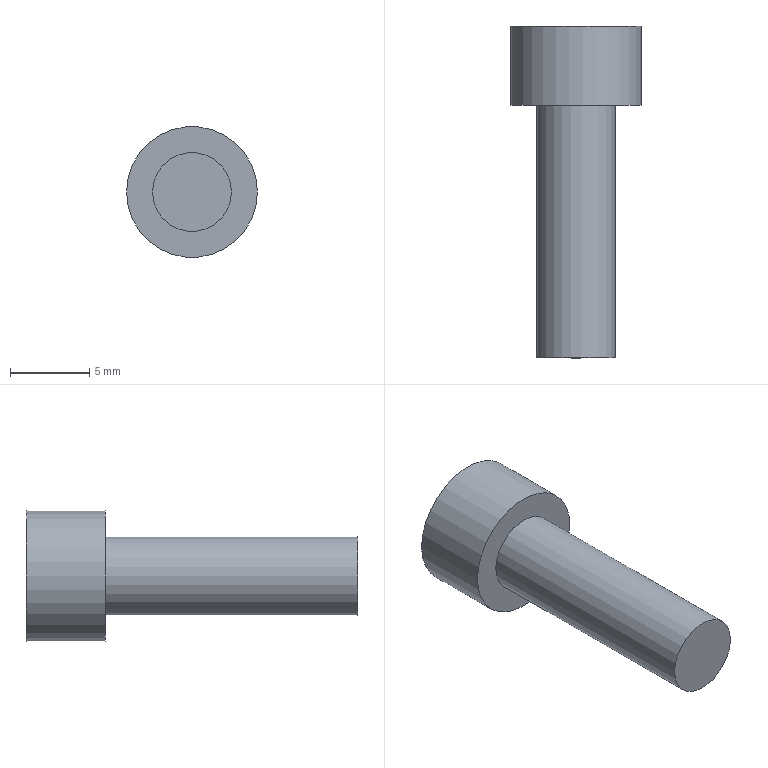Component | NX | HEX_SCREW_M5_16 | 1 solid | 12 faces | box 8.28 x 21 x 8.28 mm | volume 549 mm3 | plane 10 | cylinder 2 | commonest cylinder face diameters 8.28 x1 5 x1
STEP:
#1=CARTESIAN_POINT('',(0.,0.,0.));
#2=DIRECTION('',(0.,0.,1.));
#3=DIRECTION('',(1.,0.,0.));
#4=AXIS2_PLACEMENT_3D('',#1,#2,#3);
#5=CARTESIAN_POINT('',(26.14,-6.7,44.));
#6=VERTEX_POINT('',#5);
#7=CARTESIAN_POINT('',(22.,-6.7,44.));
#8=DIRECTION('',(0.,1.,0.));
#9=DIRECTION('',(1.,0.,0.));
#10=AXIS2_PLACEMENT_3D('',#7,#8,#9);
#11=CIRCLE('',#10,4.14);
#12=CARTESIAN_POINT('',(22.,-6.7,44.));
#13=DIRECTION('',(0.,1.,0.));
#14=DIRECTION('',(-1.,0.,0.));
#15=AXIS2_PLACEMENT_3D('',#12,#13,#14);
#16=PLANE('',#15);
#17=CARTESIAN_POINT('',(0.,0.));
#18=DIRECTION('',(-1.,0.));
#19=AXIS2_PLACEMENT_2D('',#17,#18);
#20=CIRCLE('',#19,4.14);
#21=(GEOMETRIC_REPRESENTATION_CONTEXT(2)PARAMETRIC_REPRESENTATION_CONTEXT()REPRESENTATION_CONTEXT('',''));
#22=DEFINITIONAL_REPRESENTATION('',(#20),#21);
#23=PCURVE('',#16,#22);
#24=CARTESIAN_POINT('',(22.,-11.7,44.));
#25=DIRECTION('',(0.,1.,0.));
#26=DIRECTION('',(-1.,0.,0.));
#27=AXIS2_PLACEMENT_3D('',#24,#25,#26);
#28=CYLINDRICAL_SURFACE('',#27,4.14);
#29=CARTESIAN_POINT('',(3.142,5.));
#30=DIRECTION('',(1.,0.));
#31=VECTOR('',#30,1.);
#32=LINE('',#29,#31);
#33=(GEOMETRIC_REPRESENTATION_CONTEXT(2)PARAMETRIC_REPRESENTATION_CONTEXT()REPRESENTATION_CONTEXT('',''));
#34=DEFINITIONAL_REPRESENTATION('',(#32),#33);
#35=PCURVE('',#28,#34);
#36=SURFACE_CURVE('',#11,(#23,#35),.PCURVE_S1.);
#37=EDGE_CURVE('',#6,#6,#36,.T.);
#38=ORIENTED_EDGE('',*,*,#37,.T.);
#39=EDGE_LOOP('',(#38));
#40=FACE_BOUND('',#39,.T.);
#41=CARTESIAN_POINT('',(22.,-6.7,41.691));
#42=VERTEX_POINT('',#41);
#43=CARTESIAN_POINT('',(24.,-6.7,42.845));
#44=VERTEX_POINT('',#43);
#45=CARTESIAN_POINT('',(22.,-6.7,41.691));
#46=DIRECTION('',(0.866,0.,0.5));
#47=VECTOR('',#46,1.);
#48=LINE('',#45,#47);
#49=CARTESIAN_POINT('',(0.,-2.309));
#50=DIRECTION('',(-0.866,0.5));
#51=VECTOR('',#50,1.);
#52=LINE('',#49,#51);
#53=(GEOMETRIC_REPRESENTATION_CONTEXT(2)PARAMETRIC_REPRESENTATION_CONTEXT()REPRESENTATION_CONTEXT('',''));
#54=DEFINITIONAL_REPRESENTATION('',(#52),#53);
#55=PCURVE('',#16,#54);
#56=CARTESIAN_POINT('',(22.,-9.2,41.691));
#57=DIRECTION('',(-0.5,0.,0.866));
#58=DIRECTION('',(-0.866,0.,-0.5));
#59=AXIS2_PLACEMENT_3D('',#56,#57,#58);
#60=PLANE('',#59);
#61=CARTESIAN_POINT('',(0.,-2.5));
#62=DIRECTION('',(-1.,0.));
#63=VECTOR('',#62,1.);
#64=LINE('',#61,#63);
#65=(GEOMETRIC_REPRESENTATION_CONTEXT(2)PARAMETRIC_REPRESENTATION_CONTEXT()REPRESENTATION_CONTEXT('',''));
#66=DEFINITIONAL_REPRESENTATION('',(#64),#65);
#67=PCURVE('',#60,#66);
#68=SURFACE_CURVE('',#48,(#55,#67),.PCURVE_S1.);
#69=EDGE_CURVE('',#42,#44,#68,.T.);
#70=ORIENTED_EDGE('',*,*,#69,.T.);
#71=CARTESIAN_POINT('',(24.,-6.7,45.155));
#72=VERTEX_POINT('',#71);
#73=CARTESIAN_POINT('',(24.,-6.7,42.845));
#74=DIRECTION('',(0.,0.,1.));
#75=VECTOR('',#74,1.);
#76=LINE('',#73,#75);
#77=CARTESIAN_POINT('',(-2.,-1.155));
#78=DIRECTION('',(0.,1.));
#79=VECTOR('',#78,1.);
#80=LINE('',#77,#79);
#81=(GEOMETRIC_REPRESENTATION_CONTEXT(2)PARAMETRIC_REPRESENTATION_CONTEXT()REPRESENTATION_CONTEXT('',''));
#82=DEFINITIONAL_REPRESENTATION('',(#80),#81);
#83=PCURVE('',#16,#82);
#84=CARTESIAN_POINT('',(24.,-9.2,42.845));
#85=DIRECTION('',(-1.,0.,0.));
#86=DIRECTION('',(0.,-1.,0.));
#87=AXIS2_PLACEMENT_3D('',#84,#85,#86);
#88=PLANE('',#87);
#89=CARTESIAN_POINT('',(-2.5,0.));
#90=DIRECTION('',(0.,1.));
#91=VECTOR('',#90,1.);
#92=LINE('',#89,#91);
#93=(GEOMETRIC_REPRESENTATION_CONTEXT(2)PARAMETRIC_REPRESENTATION_CONTEXT()REPRESENTATION_CONTEXT('',''));
#94=DEFINITIONAL_REPRESENTATION('',(#92),#93);
#95=PCURVE('',#88,#94);
#96=SURFACE_CURVE('',#76,(#83,#95),.PCURVE_S1.);
#97=EDGE_CURVE('',#44,#72,#96,.T.);
#98=ORIENTED_EDGE('',*,*,#97,.T.);
#99=CARTESIAN_POINT('',(22.,-6.7,46.309));
#100=VERTEX_POINT('',#99);
#101=CARTESIAN_POINT('',(24.,-6.7,45.155));
#102=DIRECTION('',(-0.866,0.,0.5));
#103=VECTOR('',#102,1.);
#104=LINE('',#101,#103);
#105=CARTESIAN_POINT('',(-2.,1.155));
#106=DIRECTION('',(0.866,0.5));
#107=VECTOR('',#106,1.);
#108=LINE('',#105,#107);
#109=(GEOMETRIC_REPRESENTATION_CONTEXT(2)PARAMETRIC_REPRESENTATION_CONTEXT()REPRESENTATION_CONTEXT('',''));
#110=DEFINITIONAL_REPRESENTATION('',(#108),#109);
#111=PCURVE('',#16,#110);
#112=CARTESIAN_POINT('',(24.,-9.2,45.155));
#113=DIRECTION('',(-0.5,0.,-0.866));
#114=DIRECTION('',(0.866,0.,-0.5));
#115=AXIS2_PLACEMENT_3D('',#112,#113,#114);
#116=PLANE('',#115);
#117=CARTESIAN_POINT('',(0.,-2.5));
#118=DIRECTION('',(-1.,0.));
#119=VECTOR('',#118,1.);
#120=LINE('',#117,#119);
#121=(GEOMETRIC_REPRESENTATION_CONTEXT(2)PARAMETRIC_REPRESENTATION_CONTEXT()REPRESENTATION_CONTEXT('',''));
#122=DEFINITIONAL_REPRESENTATION('',(#120),#121);
#123=PCURVE('',#116,#122);
#124=SURFACE_CURVE('',#104,(#111,#123),.PCURVE_S1.);
#125=EDGE_CURVE('',#72,#100,#124,.T.);
#126=ORIENTED_EDGE('',*,*,#125,.T.);
#127=CARTESIAN_POINT('',(20.,-6.7,45.155));
#128=VERTEX_POINT('',#127);
#129=CARTESIAN_POINT('',(22.,-6.7,46.309));
#130=DIRECTION('',(-0.866,0.,-0.5));
#131=VECTOR('',#130,1.);
#132=LINE('',#129,#131);
#133=CARTESIAN_POINT('',(0.,2.309));
#134=DIRECTION('',(0.866,-0.5));
#135=VECTOR('',#134,1.);
#136=LINE('',#133,#135);
#137=(GEOMETRIC_REPRESENTATION_CONTEXT(2)PARAMETRIC_REPRESENTATION_CONTEXT()REPRESENTATION_CONTEXT('',''));
#138=DEFINITIONAL_REPRESENTATION('',(#136),#137);
#139=PCURVE('',#16,#138);
#140=CARTESIAN_POINT('',(22.,-9.2,46.309));
#141=DIRECTION('',(0.5,0.,-0.866));
#142=DIRECTION('',(0.866,0.,0.5));
#143=AXIS2_PLACEMENT_3D('',#140,#141,#142);
#144=PLANE('',#143);
#145=CARTESIAN_POINT('',(0.,-2.5));
#146=DIRECTION('',(-1.,0.));
#147=VECTOR('',#146,1.);
#148=LINE('',#145,#147);
#149=(GEOMETRIC_REPRESENTATION_CONTEXT(2)PARAMETRIC_REPRESENTATION_CONTEXT()REPRESENTATION_CONTEXT('',''));
#150=DEFINITIONAL_REPRESENTATION('',(#148),#149);
#151=PCURVE('',#144,#150);
#152=SURFACE_CURVE('',#132,(#139,#151),.PCURVE_S1.);
#153=EDGE_CURVE('',#100,#128,#152,.T.);
#154=ORIENTED_EDGE('',*,*,#153,.T.);
#155=CARTESIAN_POINT('',(20.,-6.7,42.845));
#156=VERTEX_POINT('',#155);
#157=CARTESIAN_POINT('',(20.,-6.7,45.155));
#158=DIRECTION('',(0.,0.,-1.));
#159=VECTOR('',#158,1.);
#160=LINE('',#157,#159);
#161=CARTESIAN_POINT('',(2.,1.155));
#162=DIRECTION('',(0.,-1.));
#163=VECTOR('',#162,1.);
#164=LINE('',#161,#163);
#165=(GEOMETRIC_REPRESENTATION_CONTEXT(2)PARAMETRIC_REPRESENTATION_CONTEXT()REPRESENTATION_CONTEXT('',''));
#166=DEFINITIONAL_REPRESENTATION('',(#164),#165);
#167=PCURVE('',#16,#166);
#168=CARTESIAN_POINT('',(20.,-9.2,45.155));
#169=DIRECTION('',(1.,0.,0.));
#170=DIRECTION('',(0.,1.,0.));
#171=AXIS2_PLACEMENT_3D('',#168,#169,#170);
#172=PLANE('',#171);
#173=CARTESIAN_POINT('',(2.5,0.));
#174=DIRECTION('',(0.,-1.));
#175=VECTOR('',#174,1.);
#176=LINE('',#173,#175);
#177=(GEOMETRIC_REPRESENTATION_CONTEXT(2)PARAMETRIC_REPRESENTATION_CONTEXT()REPRESENTATION_CONTEXT('',''));
#178=DEFINITIONAL_REPRESENTATION('',(#176),#177);
#179=PCURVE('',#172,#178);
#180=SURFACE_CURVE('',#160,(#167,#179),.PCURVE_S1.);
#181=EDGE_CURVE('',#128,#156,#180,.T.);
#182=ORIENTED_EDGE('',*,*,#181,.T.);
#183=CARTESIAN_POINT('',(20.,-6.7,42.845));
#184=DIRECTION('',(0.866,0.,-0.5));
#185=VECTOR('',#184,1.);
#186=LINE('',#183,#185);
#187=CARTESIAN_POINT('',(2.,-1.155));
#188=DIRECTION('',(-0.866,-0.5));
#189=VECTOR('',#188,1.);
#190=LINE('',#187,#189);
#191=(GEOMETRIC_REPRESENTATION_CONTEXT(2)PARAMETRIC_REPRESENTATION_CONTEXT()REPRESENTATION_CONTEXT('',''));
#192=DEFINITIONAL_REPRESENTATION('',(#190),#191);
#193=PCURVE('',#16,#192);
#194=CARTESIAN_POINT('',(20.,-9.2,42.845));
#195=DIRECTION('',(0.5,0.,0.866));
#196=DIRECTION('',(-0.866,0.,0.5));
#197=AXIS2_PLACEMENT_3D('',#194,#195,#196);
#198=PLANE('',#197);
#199=CARTESIAN_POINT('',(0.,-2.5));
#200=DIRECTION('',(-1.,0.));
#201=VECTOR('',#200,1.);
#202=LINE('',#199,#201);
#203=(GEOMETRIC_REPRESENTATION_CONTEXT(2)PARAMETRIC_REPRESENTATION_CONTEXT()REPRESENTATION_CONTEXT('',''));
#204=DEFINITIONAL_REPRESENTATION('',(#202),#203);
#205=PCURVE('',#198,#204);
#206=SURFACE_CURVE('',#186,(#193,#205),.PCURVE_S1.);
#207=EDGE_CURVE('',#156,#42,#206,.T.);
#208=ORIENTED_EDGE('',*,*,#207,.T.);
#209=EDGE_LOOP('',(#70,#98,#126,#154,#182,#208));
#210=FACE_BOUND('',#209,.T.);
#211=ADVANCED_FACE('',(#40,#210),#16,.T.);
#212=CARTESIAN_POINT('',(26.14,-11.7,44.));
#213=VERTEX_POINT('',#212);
#214=CARTESIAN_POINT('',(22.,-11.7,44.));
#215=DIRECTION('',(0.,1.,0.));
#216=DIRECTION('',(1.,0.,0.));
#217=AXIS2_PLACEMENT_3D('',#214,#215,#216);
#218=CIRCLE('',#217,4.14);
#219=CARTESIAN_POINT('',(3.142,0.));
#220=DIRECTION('',(1.,0.));
#221=VECTOR('',#220,1.);
#222=LINE('',#219,#221);
#223=(GEOMETRIC_REPRESENTATION_CONTEXT(2)PARAMETRIC_REPRESENTATION_CONTEXT()REPRESENTATION_CONTEXT('',''));
#224=DEFINITIONAL_REPRESENTATION('',(#222),#223);
#225=PCURVE('',#28,#224);
#226=CARTESIAN_POINT('',(22.,-11.7,44.));
#227=DIRECTION('',(0.,1.,0.));
#228=DIRECTION('',(-1.,0.,0.));
#229=AXIS2_PLACEMENT_3D('',#226,#227,#228);
#230=PLANE('',#229);
#231=CARTESIAN_POINT('',(0.,0.));
#232=DIRECTION('',(-1.,0.));
#233=AXIS2_PLACEMENT_2D('',#231,#232);
#234=CIRCLE('',#233,4.14);
#235=(GEOMETRIC_REPRESENTATION_CONTEXT(2)PARAMETRIC_REPRESENTATION_CONTEXT()REPRESENTATION_CONTEXT('',''));
#236=DEFINITIONAL_REPRESENTATION('',(#234),#235);
#237=PCURVE('',#230,#236);
#238=SURFACE_CURVE('',#218,(#225,#237),.PCURVE_S1.);
#239=EDGE_CURVE('',#213,#213,#238,.T.);
#240=ORIENTED_EDGE('',*,*,#239,.T.);
#241=CARTESIAN_POINT('',(26.14,-11.7,44.));
#242=CARTESIAN_POINT('',(26.14,-6.7,44.));
#243=B_SPLINE_CURVE_WITH_KNOTS('',1,(#241,#242),.UNSPECIFIED.,.F.,.F.,(2,2),(0.,5.),.PIECEWISE_BEZIER_KNOTS.);
#244=CARTESIAN_POINT('',(9.425,0.));
#245=DIRECTION('',(0.,1.));
#246=VECTOR('',#245,1.);
#247=LINE('',#244,#246);
#248=(GEOMETRIC_REPRESENTATION_CONTEXT(2)PARAMETRIC_REPRESENTATION_CONTEXT()REPRESENTATION_CONTEXT('',''));
#249=DEFINITIONAL_REPRESENTATION('',(#247),#248);
#250=PCURVE('',#28,#249);
#251=CARTESIAN_POINT('',(3.142,0.));
#252=DIRECTION('',(0.,1.));
#253=VECTOR('',#252,1.);
#254=LINE('',#251,#253);
#255=(GEOMETRIC_REPRESENTATION_CONTEXT(2)PARAMETRIC_REPRESENTATION_CONTEXT()REPRESENTATION_CONTEXT('',''));
#256=DEFINITIONAL_REPRESENTATION('',(#254),#255);
#257=PCURVE('',#28,#256);
#258=SEAM_CURVE('',#243,(#250,#257),.PCURVE_S1.);
#259=EDGE_CURVE('',#213,#6,#258,.T.);
#260=ORIENTED_EDGE('',*,*,#259,.T.);
#261=ORIENTED_EDGE('',*,*,#37,.F.);
#262=ORIENTED_EDGE('',*,*,#259,.F.);
#263=EDGE_LOOP('',(#240,#260,#261,#262));
#264=FACE_BOUND('',#263,.T.);
#265=ADVANCED_FACE('',(#264),#28,.T.);
#266=CARTESIAN_POINT('',(24.5,-11.7,44.));
#267=VERTEX_POINT('',#266);
#268=CARTESIAN_POINT('',(22.,-11.7,44.));
#269=DIRECTION('',(0.,1.,0.));
#270=DIRECTION('',(1.,0.,0.));
#271=AXIS2_PLACEMENT_3D('',#268,#269,#270);
#272=CIRCLE('',#271,2.5);
#273=CARTESIAN_POINT('',(0.,0.));
#274=DIRECTION('',(-1.,0.));
#275=AXIS2_PLACEMENT_2D('',#273,#274);
#276=CIRCLE('',#275,2.5);
#277=(GEOMETRIC_REPRESENTATION_CONTEXT(2)PARAMETRIC_REPRESENTATION_CONTEXT()REPRESENTATION_CONTEXT('',''));
#278=DEFINITIONAL_REPRESENTATION('',(#276),#277);
#279=PCURVE('',#230,#278);
#280=CARTESIAN_POINT('',(22.,-27.7,44.));
#281=DIRECTION('',(0.,1.,0.));
#282=DIRECTION('',(-1.,0.,0.));
#283=AXIS2_PLACEMENT_3D('',#280,#281,#282);
#284=CYLINDRICAL_SURFACE('',#283,2.5);
#285=CARTESIAN_POINT('',(3.142,16.));
#286=DIRECTION('',(1.,0.));
#287=VECTOR('',#286,1.);
#288=LINE('',#285,#287);
#289=(GEOMETRIC_REPRESENTATION_CONTEXT(2)PARAMETRIC_REPRESENTATION_CONTEXT()REPRESENTATION_CONTEXT('',''));
#290=DEFINITIONAL_REPRESENTATION('',(#288),#289);
#291=PCURVE('',#284,#290);
#292=SURFACE_CURVE('',#272,(#279,#291),.PCURVE_S1.);
#293=EDGE_CURVE('',#267,#267,#292,.T.);
#294=ORIENTED_EDGE('',*,*,#293,.T.);
#295=EDGE_LOOP('',(#294));
#296=FACE_BOUND('',#295,.T.);
#297=ORIENTED_EDGE('',*,*,#239,.F.);
#298=EDGE_LOOP('',(#297));
#299=FACE_BOUND('',#298,.T.);
#300=ADVANCED_FACE('',(#296,#299),#230,.F.);
#301=CARTESIAN_POINT('',(24.5,-27.7,44.));
#302=VERTEX_POINT('',#301);
#303=CARTESIAN_POINT('',(22.,-27.7,44.));
#304=DIRECTION('',(0.,1.,0.));
#305=DIRECTION('',(1.,0.,0.));
#306=AXIS2_PLACEMENT_3D('',#303,#304,#305);
#307=CIRCLE('',#306,2.5);
#308=CARTESIAN_POINT('',(3.142,0.));
#309=DIRECTION('',(1.,0.));
#310=VECTOR('',#309,1.);
#311=LINE('',#308,#310);
#312=(GEOMETRIC_REPRESENTATION_CONTEXT(2)PARAMETRIC_REPRESENTATION_CONTEXT()REPRESENTATION_CONTEXT('',''));
#313=DEFINITIONAL_REPRESENTATION('',(#311),#312);
#314=PCURVE('',#284,#313);
#315=CARTESIAN_POINT('',(22.,-27.7,44.));
#316=DIRECTION('',(0.,1.,0.));
#317=DIRECTION('',(-1.,0.,0.));
#318=AXIS2_PLACEMENT_3D('',#315,#316,#317);
#319=PLANE('',#318);
#320=CARTESIAN_POINT('',(0.,0.));
#321=DIRECTION('',(-1.,0.));
#322=AXIS2_PLACEMENT_2D('',#320,#321);
#323=CIRCLE('',#322,2.5);
#324=(GEOMETRIC_REPRESENTATION_CONTEXT(2)PARAMETRIC_REPRESENTATION_CONTEXT()REPRESENTATION_CONTEXT('',''));
#325=DEFINITIONAL_REPRESENTATION('',(#323),#324);
#326=PCURVE('',#319,#325);
#327=SURFACE_CURVE('',#307,(#314,#326),.PCURVE_S1.);
#328=EDGE_CURVE('',#302,#302,#327,.T.);
#329=ORIENTED_EDGE('',*,*,#328,.T.);
#330=CARTESIAN_POINT('',(24.5,-27.7,44.));
#331=CARTESIAN_POINT('',(24.5,-11.7,44.));
#332=B_SPLINE_CURVE_WITH_KNOTS('',1,(#330,#331),.UNSPECIFIED.,.F.,.F.,(2,2),(0.,16.),.PIECEWISE_BEZIER_KNOTS.);
#333=CARTESIAN_POINT('',(9.425,0.));
#334=DIRECTION('',(0.,1.));
#335=VECTOR('',#334,1.);
#336=LINE('',#333,#335);
#337=(GEOMETRIC_REPRESENTATION_CONTEXT(2)PARAMETRIC_REPRESENTATION_CONTEXT()REPRESENTATION_CONTEXT('',''));
#338=DEFINITIONAL_REPRESENTATION('',(#336),#337);
#339=PCURVE('',#284,#338);
#340=CARTESIAN_POINT('',(3.142,0.));
#341=DIRECTION('',(0.,1.));
#342=VECTOR('',#341,1.);
#343=LINE('',#340,#342);
#344=(GEOMETRIC_REPRESENTATION_CONTEXT(2)PARAMETRIC_REPRESENTATION_CONTEXT()REPRESENTATION_CONTEXT('',''));
#345=DEFINITIONAL_REPRESENTATION('',(#343),#344);
#346=PCURVE('',#284,#345);
#347=SEAM_CURVE('',#332,(#339,#346),.PCURVE_S1.);
#348=EDGE_CURVE('',#302,#267,#347,.T.);
#349=ORIENTED_EDGE('',*,*,#348,.T.);
#350=ORIENTED_EDGE('',*,*,#293,.F.);
#351=ORIENTED_EDGE('',*,*,#348,.F.);
#352=EDGE_LOOP('',(#329,#349,#350,#351));
#353=FACE_BOUND('',#352,.T.);
#354=ADVANCED_FACE('',(#353),#284,.T.);
#355=ORIENTED_EDGE('',*,*,#328,.F.);
#356=EDGE_LOOP('',(#355));
#357=FACE_BOUND('',#356,.T.);
#358=ADVANCED_FACE('',(#357),#319,.F.);
#359=ORIENTED_EDGE('',*,*,#97,.F.);
#360=CARTESIAN_POINT('',(24.,-9.2,42.845));
#361=VERTEX_POINT('',#360);
#362=CARTESIAN_POINT('',(24.,-9.2,42.845));
#363=DIRECTION('',(0.,-1.,0.));
#364=VECTOR('',#363,1.);
#365=LINE('',#362,#364);
#366=CARTESIAN_POINT('',(0.,0.));
#367=DIRECTION('',(1.,0.));
#368=VECTOR('',#367,1.);
#369=LINE('',#366,#368);
#370=(GEOMETRIC_REPRESENTATION_CONTEXT(2)PARAMETRIC_REPRESENTATION_CONTEXT()REPRESENTATION_CONTEXT('',''));
#371=DEFINITIONAL_REPRESENTATION('',(#369),#370);
#372=PCURVE('',#88,#371);
#373=CARTESIAN_POINT('',(-2.309,0.));
#374=DIRECTION('',(0.,1.));
#375=VECTOR('',#374,1.);
#376=LINE('',#373,#375);
#377=(GEOMETRIC_REPRESENTATION_CONTEXT(2)PARAMETRIC_REPRESENTATION_CONTEXT()REPRESENTATION_CONTEXT('',''));
#378=DEFINITIONAL_REPRESENTATION('',(#376),#377);
#379=PCURVE('',#60,#378);
#380=SURFACE_CURVE('',#365,(#372,#379),.PCURVE_S1.);
#381=EDGE_CURVE('',#44,#361,#380,.T.);
#382=ORIENTED_EDGE('',*,*,#381,.T.);
#383=CARTESIAN_POINT('',(24.,-9.2,45.155));
#384=VERTEX_POINT('',#383);
#385=CARTESIAN_POINT('',(24.,-9.2,42.845));
#386=DIRECTION('',(0.,0.,-1.));
#387=VECTOR('',#386,1.);
#388=LINE('',#385,#387);
#389=CARTESIAN_POINT('',(0.,0.));
#390=DIRECTION('',(0.,-1.));
#391=VECTOR('',#390,1.);
#392=LINE('',#389,#391);
#393=(GEOMETRIC_REPRESENTATION_CONTEXT(2)PARAMETRIC_REPRESENTATION_CONTEXT()REPRESENTATION_CONTEXT('',''));
#394=DEFINITIONAL_REPRESENTATION('',(#392),#393);
#395=PCURVE('',#88,#394);
#396=CARTESIAN_POINT('',(22.,-9.2,44.));
#397=DIRECTION('',(0.,-1.,0.));
#398=DIRECTION('',(1.,0.,0.));
#399=AXIS2_PLACEMENT_3D('',#396,#397,#398);
#400=PLANE('',#399);
#401=CARTESIAN_POINT('',(2.,-1.155));
#402=DIRECTION('',(0.,-1.));
#403=VECTOR('',#402,1.);
#404=LINE('',#401,#403);
#405=(GEOMETRIC_REPRESENTATION_CONTEXT(2)PARAMETRIC_REPRESENTATION_CONTEXT()REPRESENTATION_CONTEXT('',''));
#406=DEFINITIONAL_REPRESENTATION('',(#404),#405);
#407=PCURVE('',#400,#406);
#408=SURFACE_CURVE('',#388,(#395,#407),.PCURVE_S1.);
#409=EDGE_CURVE('',#384,#361,#408,.T.);
#410=ORIENTED_EDGE('',*,*,#409,.F.);
#411=CARTESIAN_POINT('',(24.,-9.2,45.155));
#412=DIRECTION('',(0.,-1.,0.));
#413=VECTOR('',#412,1.);
#414=LINE('',#411,#413);
#415=CARTESIAN_POINT('',(0.,2.309));
#416=DIRECTION('',(1.,0.));
#417=VECTOR('',#416,1.);
#418=LINE('',#415,#417);
#419=(GEOMETRIC_REPRESENTATION_CONTEXT(2)PARAMETRIC_REPRESENTATION_CONTEXT()REPRESENTATION_CONTEXT('',''));
#420=DEFINITIONAL_REPRESENTATION('',(#418),#419);
#421=PCURVE('',#88,#420);
#422=CARTESIAN_POINT('',(0.,0.));
#423=DIRECTION('',(0.,1.));
#424=VECTOR('',#423,1.);
#425=LINE('',#422,#424);
#426=(GEOMETRIC_REPRESENTATION_CONTEXT(2)PARAMETRIC_REPRESENTATION_CONTEXT()REPRESENTATION_CONTEXT('',''));
#427=DEFINITIONAL_REPRESENTATION('',(#425),#426);
#428=PCURVE('',#116,#427);
#429=SURFACE_CURVE('',#414,(#421,#428),.PCURVE_S1.);
#430=EDGE_CURVE('',#72,#384,#429,.T.);
#431=ORIENTED_EDGE('',*,*,#430,.F.);
#432=EDGE_LOOP('',(#359,#382,#410,#431));
#433=FACE_BOUND('',#432,.T.);
#434=ADVANCED_FACE('',(#433),#88,.T.);
#435=ORIENTED_EDGE('',*,*,#125,.F.);
#436=ORIENTED_EDGE('',*,*,#430,.T.);
#437=CARTESIAN_POINT('',(22.,-9.2,46.309));
#438=VERTEX_POINT('',#437);
#439=CARTESIAN_POINT('',(24.,-9.2,45.155));
#440=DIRECTION('',(0.866,0.,-0.5));
#441=VECTOR('',#440,1.);
#442=LINE('',#439,#441);
#443=CARTESIAN_POINT('',(0.,0.));
#444=DIRECTION('',(1.,0.));
#445=VECTOR('',#444,1.);
#446=LINE('',#443,#445);
#447=(GEOMETRIC_REPRESENTATION_CONTEXT(2)PARAMETRIC_REPRESENTATION_CONTEXT()REPRESENTATION_CONTEXT('',''));
#448=DEFINITIONAL_REPRESENTATION('',(#446),#447);
#449=PCURVE('',#116,#448);
#450=CARTESIAN_POINT('',(2.,1.155));
#451=DIRECTION('',(0.866,-0.5));
#452=VECTOR('',#451,1.);
#453=LINE('',#450,#452);
#454=(GEOMETRIC_REPRESENTATION_CONTEXT(2)PARAMETRIC_REPRESENTATION_CONTEXT()REPRESENTATION_CONTEXT('',''));
#455=DEFINITIONAL_REPRESENTATION('',(#453),#454);
#456=PCURVE('',#400,#455);
#457=SURFACE_CURVE('',#442,(#449,#456),.PCURVE_S1.);
#458=EDGE_CURVE('',#438,#384,#457,.T.);
#459=ORIENTED_EDGE('',*,*,#458,.F.);
#460=CARTESIAN_POINT('',(22.,-9.2,46.309));
#461=DIRECTION('',(0.,-1.,0.));
#462=VECTOR('',#461,1.);
#463=LINE('',#460,#462);
#464=CARTESIAN_POINT('',(-2.309,0.));
#465=DIRECTION('',(0.,1.));
#466=VECTOR('',#465,1.);
#467=LINE('',#464,#466);
#468=(GEOMETRIC_REPRESENTATION_CONTEXT(2)PARAMETRIC_REPRESENTATION_CONTEXT()REPRESENTATION_CONTEXT('',''));
#469=DEFINITIONAL_REPRESENTATION('',(#467),#468);
#470=PCURVE('',#116,#469);
#471=CARTESIAN_POINT('',(0.,0.));
#472=DIRECTION('',(0.,1.));
#473=VECTOR('',#472,1.);
#474=LINE('',#471,#473);
#475=(GEOMETRIC_REPRESENTATION_CONTEXT(2)PARAMETRIC_REPRESENTATION_CONTEXT()REPRESENTATION_CONTEXT('',''));
#476=DEFINITIONAL_REPRESENTATION('',(#474),#475);
#477=PCURVE('',#144,#476);
#478=SURFACE_CURVE('',#463,(#470,#477),.PCURVE_S1.);
#479=EDGE_CURVE('',#100,#438,#478,.T.);
#480=ORIENTED_EDGE('',*,*,#479,.F.);
#481=EDGE_LOOP('',(#435,#436,#459,#480));
#482=FACE_BOUND('',#481,.T.);
#483=ADVANCED_FACE('',(#482),#116,.T.);
#484=ORIENTED_EDGE('',*,*,#153,.F.);
#485=ORIENTED_EDGE('',*,*,#479,.T.);
#486=CARTESIAN_POINT('',(20.,-9.2,45.155));
#487=VERTEX_POINT('',#486);
#488=CARTESIAN_POINT('',(22.,-9.2,46.309));
#489=DIRECTION('',(0.866,0.,0.5));
#490=VECTOR('',#489,1.);
#491=LINE('',#488,#490);
#492=CARTESIAN_POINT('',(0.,0.));
#493=DIRECTION('',(1.,0.));
#494=VECTOR('',#493,1.);
#495=LINE('',#492,#494);
#496=(GEOMETRIC_REPRESENTATION_CONTEXT(2)PARAMETRIC_REPRESENTATION_CONTEXT()REPRESENTATION_CONTEXT('',''));
#497=DEFINITIONAL_REPRESENTATION('',(#495),#496);
#498=PCURVE('',#144,#497);
#499=CARTESIAN_POINT('',(0.,2.309));
#500=DIRECTION('',(0.866,0.5));
#501=VECTOR('',#500,1.);
#502=LINE('',#499,#501);
#503=(GEOMETRIC_REPRESENTATION_CONTEXT(2)PARAMETRIC_REPRESENTATION_CONTEXT()REPRESENTATION_CONTEXT('',''));
#504=DEFINITIONAL_REPRESENTATION('',(#502),#503);
#505=PCURVE('',#400,#504);
#506=SURFACE_CURVE('',#491,(#498,#505),.PCURVE_S1.);
#507=EDGE_CURVE('',#487,#438,#506,.T.);
#508=ORIENTED_EDGE('',*,*,#507,.F.);
#509=CARTESIAN_POINT('',(20.,-9.2,45.155));
#510=DIRECTION('',(0.,-1.,0.));
#511=VECTOR('',#510,1.);
#512=LINE('',#509,#511);
#513=CARTESIAN_POINT('',(-2.309,0.));
#514=DIRECTION('',(0.,1.));
#515=VECTOR('',#514,1.);
#516=LINE('',#513,#515);
#517=(GEOMETRIC_REPRESENTATION_CONTEXT(2)PARAMETRIC_REPRESENTATION_CONTEXT()REPRESENTATION_CONTEXT('',''));
#518=DEFINITIONAL_REPRESENTATION('',(#516),#517);
#519=PCURVE('',#144,#518);
#520=CARTESIAN_POINT('',(0.,0.));
#521=DIRECTION('',(-1.,0.));
#522=VECTOR('',#521,1.);
#523=LINE('',#520,#522);
#524=(GEOMETRIC_REPRESENTATION_CONTEXT(2)PARAMETRIC_REPRESENTATION_CONTEXT()REPRESENTATION_CONTEXT('',''));
#525=DEFINITIONAL_REPRESENTATION('',(#523),#524);
#526=PCURVE('',#172,#525);
#527=SURFACE_CURVE('',#512,(#519,#526),.PCURVE_S1.);
#528=EDGE_CURVE('',#128,#487,#527,.T.);
#529=ORIENTED_EDGE('',*,*,#528,.F.);
#530=EDGE_LOOP('',(#484,#485,#508,#529));
#531=FACE_BOUND('',#530,.T.);
#532=ADVANCED_FACE('',(#531),#144,.T.);
#533=ORIENTED_EDGE('',*,*,#181,.F.);
#534=ORIENTED_EDGE('',*,*,#528,.T.);
#535=CARTESIAN_POINT('',(20.,-9.2,42.845));
#536=VERTEX_POINT('',#535);
#537=CARTESIAN_POINT('',(20.,-9.2,45.155));
#538=DIRECTION('',(0.,0.,1.));
#539=VECTOR('',#538,1.);
#540=LINE('',#537,#539);
#541=CARTESIAN_POINT('',(0.,0.));
#542=DIRECTION('',(0.,1.));
#543=VECTOR('',#542,1.);
#544=LINE('',#541,#543);
#545=(GEOMETRIC_REPRESENTATION_CONTEXT(2)PARAMETRIC_REPRESENTATION_CONTEXT()REPRESENTATION_CONTEXT('',''));
#546=DEFINITIONAL_REPRESENTATION('',(#544),#545);
#547=PCURVE('',#172,#546);
#548=CARTESIAN_POINT('',(-2.,1.155));
#549=DIRECTION('',(0.,1.));
#550=VECTOR('',#549,1.);
#551=LINE('',#548,#550);
#552=(GEOMETRIC_REPRESENTATION_CONTEXT(2)PARAMETRIC_REPRESENTATION_CONTEXT()REPRESENTATION_CONTEXT('',''));
#553=DEFINITIONAL_REPRESENTATION('',(#551),#552);
#554=PCURVE('',#400,#553);
#555=SURFACE_CURVE('',#540,(#547,#554),.PCURVE_S1.);
#556=EDGE_CURVE('',#536,#487,#555,.T.);
#557=ORIENTED_EDGE('',*,*,#556,.F.);
#558=CARTESIAN_POINT('',(20.,-9.2,42.845));
#559=DIRECTION('',(0.,-1.,0.));
#560=VECTOR('',#559,1.);
#561=LINE('',#558,#560);
#562=CARTESIAN_POINT('',(0.,-2.309));
#563=DIRECTION('',(-1.,0.));
#564=VECTOR('',#563,1.);
#565=LINE('',#562,#564);
#566=(GEOMETRIC_REPRESENTATION_CONTEXT(2)PARAMETRIC_REPRESENTATION_CONTEXT()REPRESENTATION_CONTEXT('',''));
#567=DEFINITIONAL_REPRESENTATION('',(#565),#566);
#568=PCURVE('',#172,#567);
#569=CARTESIAN_POINT('',(0.,0.));
#570=DIRECTION('',(0.,1.));
#571=VECTOR('',#570,1.);
#572=LINE('',#569,#571);
#573=(GEOMETRIC_REPRESENTATION_CONTEXT(2)PARAMETRIC_REPRESENTATION_CONTEXT()REPRESENTATION_CONTEXT('',''));
#574=DEFINITIONAL_REPRESENTATION('',(#572),#573);
#575=PCURVE('',#198,#574);
#576=SURFACE_CURVE('',#561,(#568,#575),.PCURVE_S1.);
#577=EDGE_CURVE('',#156,#536,#576,.T.);
#578=ORIENTED_EDGE('',*,*,#577,.F.);
#579=EDGE_LOOP('',(#533,#534,#557,#578));
#580=FACE_BOUND('',#579,.T.);
#581=ADVANCED_FACE('',(#580),#172,.T.);
#582=ORIENTED_EDGE('',*,*,#207,.F.);
#583=ORIENTED_EDGE('',*,*,#577,.T.);
#584=CARTESIAN_POINT('',(22.,-9.2,41.691));
#585=VERTEX_POINT('',#584);
#586=CARTESIAN_POINT('',(20.,-9.2,42.845));
#587=DIRECTION('',(-0.866,0.,0.5));
#588=VECTOR('',#587,1.);
#589=LINE('',#586,#588);
#590=CARTESIAN_POINT('',(0.,0.));
#591=DIRECTION('',(1.,0.));
#592=VECTOR('',#591,1.);
#593=LINE('',#590,#592);
#594=(GEOMETRIC_REPRESENTATION_CONTEXT(2)PARAMETRIC_REPRESENTATION_CONTEXT()REPRESENTATION_CONTEXT('',''));
#595=DEFINITIONAL_REPRESENTATION('',(#593),#594);
#596=PCURVE('',#198,#595);
#597=CARTESIAN_POINT('',(-2.,-1.155));
#598=DIRECTION('',(-0.866,0.5));
#599=VECTOR('',#598,1.);
#600=LINE('',#597,#599);
#601=(GEOMETRIC_REPRESENTATION_CONTEXT(2)PARAMETRIC_REPRESENTATION_CONTEXT()REPRESENTATION_CONTEXT('',''));
#602=DEFINITIONAL_REPRESENTATION('',(#600),#601);
#603=PCURVE('',#400,#602);
#604=SURFACE_CURVE('',#589,(#596,#603),.PCURVE_S1.);
#605=EDGE_CURVE('',#585,#536,#604,.T.);
#606=ORIENTED_EDGE('',*,*,#605,.F.);
#607=CARTESIAN_POINT('',(22.,-9.2,41.691));
#608=DIRECTION('',(0.,-1.,0.));
#609=VECTOR('',#608,1.);
#610=LINE('',#607,#609);
#611=CARTESIAN_POINT('',(-2.309,0.));
#612=DIRECTION('',(0.,1.));
#613=VECTOR('',#612,1.);
#614=LINE('',#611,#613);
#615=(GEOMETRIC_REPRESENTATION_CONTEXT(2)PARAMETRIC_REPRESENTATION_CONTEXT()REPRESENTATION_CONTEXT('',''));
#616=DEFINITIONAL_REPRESENTATION('',(#614),#615);
#617=PCURVE('',#198,#616);
#618=CARTESIAN_POINT('',(0.,0.));
#619=DIRECTION('',(0.,1.));
#620=VECTOR('',#619,1.);
#621=LINE('',#618,#620);
#622=(GEOMETRIC_REPRESENTATION_CONTEXT(2)PARAMETRIC_REPRESENTATION_CONTEXT()REPRESENTATION_CONTEXT('',''));
#623=DEFINITIONAL_REPRESENTATION('',(#621),#622);
#624=PCURVE('',#60,#623);
#625=SURFACE_CURVE('',#610,(#617,#624),.PCURVE_S1.);
#626=EDGE_CURVE('',#42,#585,#625,.T.);
#627=ORIENTED_EDGE('',*,*,#626,.F.);
#628=EDGE_LOOP('',(#582,#583,#606,#627));
#629=FACE_BOUND('',#628,.T.);
#630=ADVANCED_FACE('',(#629),#198,.T.);
#631=ORIENTED_EDGE('',*,*,#69,.F.);
#632=ORIENTED_EDGE('',*,*,#626,.T.);
#633=CARTESIAN_POINT('',(22.,-9.2,41.691));
#634=DIRECTION('',(-0.866,0.,-0.5));
#635=VECTOR('',#634,1.);
#636=LINE('',#633,#635);
#637=CARTESIAN_POINT('',(0.,0.));
#638=DIRECTION('',(1.,0.));
#639=VECTOR('',#638,1.);
#640=LINE('',#637,#639);
#641=(GEOMETRIC_REPRESENTATION_CONTEXT(2)PARAMETRIC_REPRESENTATION_CONTEXT()REPRESENTATION_CONTEXT('',''));
#642=DEFINITIONAL_REPRESENTATION('',(#640),#641);
#643=PCURVE('',#60,#642);
#644=CARTESIAN_POINT('',(0.,-2.309));
#645=DIRECTION('',(-0.866,-0.5));
#646=VECTOR('',#645,1.);
#647=LINE('',#644,#646);
#648=(GEOMETRIC_REPRESENTATION_CONTEXT(2)PARAMETRIC_REPRESENTATION_CONTEXT()REPRESENTATION_CONTEXT('',''));
#649=DEFINITIONAL_REPRESENTATION('',(#647),#648);
#650=PCURVE('',#400,#649);
#651=SURFACE_CURVE('',#636,(#643,#650),.PCURVE_S1.);
#652=EDGE_CURVE('',#361,#585,#651,.T.);
#653=ORIENTED_EDGE('',*,*,#652,.F.);
#654=ORIENTED_EDGE('',*,*,#381,.F.);
#655=EDGE_LOOP('',(#631,#632,#653,#654));
#656=FACE_BOUND('',#655,.T.);
#657=ADVANCED_FACE('',(#656),#60,.T.);
#658=ORIENTED_EDGE('',*,*,#409,.T.);
#659=ORIENTED_EDGE('',*,*,#652,.T.);
#660=ORIENTED_EDGE('',*,*,#605,.T.);
#661=ORIENTED_EDGE('',*,*,#556,.T.);
#662=ORIENTED_EDGE('',*,*,#507,.T.);
#663=ORIENTED_EDGE('',*,*,#458,.T.);
#664=EDGE_LOOP('',(#658,#659,#660,#661,#662,#663));
#665=FACE_BOUND('',#664,.T.);
#666=ADVANCED_FACE('',(#665),#400,.F.);
#667=CLOSED_SHELL('',(#211,#265,#300,#354,#358,#434,#483,#532,#581,#630,#657,#666));
#668=MANIFOLD_SOLID_BREP('',#667);
#669=(LENGTH_UNIT()NAMED_UNIT(*)SI_UNIT(.MILLI.,.METRE.));
#670=UNCERTAINTY_MEASURE_WITH_UNIT(LENGTH_MEASURE(0.000002),#669,'','');
#671=(NAMED_UNIT(*)PLANE_ANGLE_UNIT()SI_UNIT($,.RADIAN.));
#672=(NAMED_UNIT(*)SI_UNIT($,.STERADIAN.)SOLID_ANGLE_UNIT());
#673=(GEOMETRIC_REPRESENTATION_CONTEXT(3)GLOBAL_UNCERTAINTY_ASSIGNED_CONTEXT((#670))GLOBAL_UNIT_ASSIGNED_CONTEXT((#669,#671,#672))REPRESENTATION_CONTEXT('',''));
#674=ADVANCED_BREP_SHAPE_REPRESENTATION('',(#4,#668),#673);